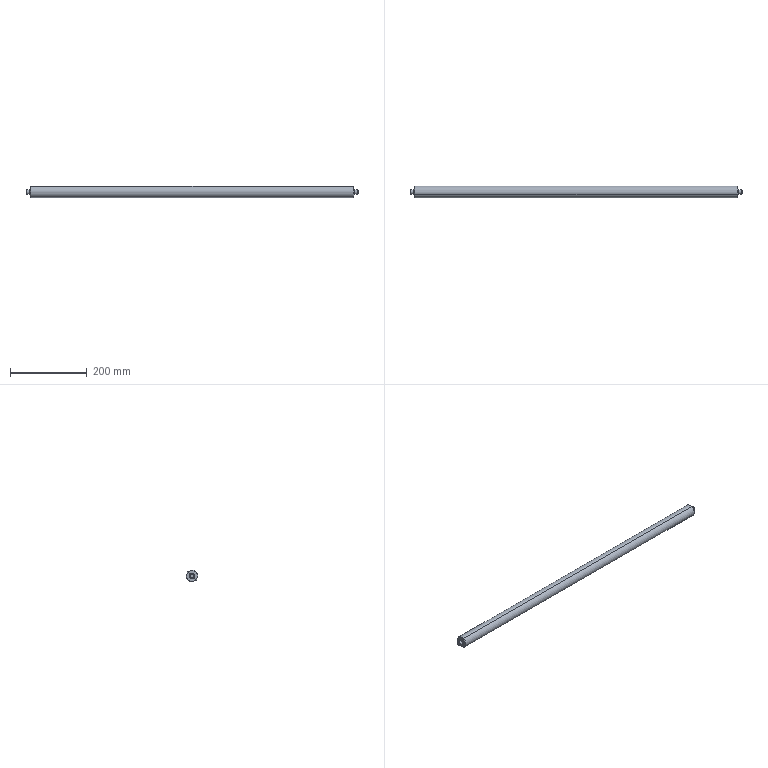Component | SolidWorks | DrivenAxis-1_MainFeedAxis1-1 | 1 solid | 28 faces | box 865 x 30 x 30 mm | volume 598579 mm3 | cone 12 | cylinder 10 | plane 6 | commonest cylinder face diameters 12 x4 15 x4 30 x2
build123d program:
from build123d import *

# Parameters (mm, degrees)
SKETCH1_R           = 15
BOSS_EXTRUDE1_DEPTH = 843
SKETCH3_R           = 7.5
BOSS_EXTRUDE2_DEPTH = 3
BOSS_EXTRUDE3_START = 3
SKETCH4_R           = 7.5
BOSS_EXTRUDE3_DEPTH = 3
SKETCH5_R           = 6
BOSS_EXTRUDE4_DEPTH = 8
BOSS_EXTRUDE5_START = 8
SKETCH6_R           = 6
BOSS_EXTRUDE5_DEPTH = 8
CHAMFER1_SIZE       = 1
CHAMFER2_SIZE       = 1


with BuildPart() as part:
    # Sketch1 → Boss-Extrude1 (new body)
    with BuildSketch(Plane.XY):
        with Locations(Location((0, 0, 0), (0, 0, 180))):
            Circle(SKETCH1_R)
    extrude(amount=BOSS_EXTRUDE1_DEPTH)

    # Sketch3 → Boss-Extrude2 (add)
    with BuildSketch(Plane.XY.offset(843)):
        Circle(SKETCH3_R)
    extrude(amount=BOSS_EXTRUDE2_DEPTH)

    # Sketch4 → Boss-Extrude3 (add)
    with BuildSketch(Plane(origin=(0, 0, 0), x_dir=(-1, 0, 0), z_dir=(0, 0, -1)).offset(BOSS_EXTRUDE3_START)):
        with Locations(Location((0, 0, 0), (0, 0, 180))):
            Circle(SKETCH4_R)
    extrude(amount=-BOSS_EXTRUDE3_DEPTH)

    # Sketch5 → Boss-Extrude4 (add)
    with BuildSketch(Plane(origin=(0, 0, -3), x_dir=(-1, 0, 0), z_dir=(0, 0, -1))):
        Circle(SKETCH5_R)
    extrude(amount=BOSS_EXTRUDE4_DEPTH)

    # Sketch6 → Boss-Extrude5 (add)
    with BuildSketch(Plane.XY.offset(846).offset(BOSS_EXTRUDE5_START)):
        with Locations(Location((0, 0, 0), (0, 0, 180))):
            Circle(SKETCH6_R)
    extrude(amount=-BOSS_EXTRUDE5_DEPTH)

    # Chamfer1
    chamfer1_edges = [part.edges().sort_by_distance(p)[0] for p in [
        (6, 0, 854),
        (15, 0, 843),
        (-7.5, 0, 846),
    ]]
    chamfer(chamfer1_edges, length=CHAMFER1_SIZE)

    # Chamfer2
    chamfer2_edges = [part.edges().sort_by_distance(p)[0] for p in [
        (-7.5, 0, -3),
        (6, 0, -11),
        (15, 0, 0),
    ]]
    chamfer(chamfer2_edges, length=CHAMFER2_SIZE)


solid = part.part

# Placed as in the assembly
solid = solid.moved(Location((13, -30, -174.268), (0, 90, 0)))
STEP:
#1=COLOUR_RGB('',0.7922,0.8196,0.9333);
#2=FILL_AREA_STYLE_COLOUR('',#1);
#3=FILL_AREA_STYLE('',(#2));
#4=SURFACE_STYLE_FILL_AREA(#3);
#5=SURFACE_SIDE_STYLE('',(#4));
#6=SURFACE_STYLE_USAGE(.BOTH.,#5);
#7=PRESENTATION_STYLE_ASSIGNMENT((#6));
#8=CARTESIAN_POINT('',(33.701,-0.9596,-7.366));
#9=VERTEX_POINT('',#8);
#10=CARTESIAN_POINT('',(33.701,-1.403,-6.356));
#11=VERTEX_POINT('',#10);
#12=CARTESIAN_POINT('',(33.701,-1.181,-6.861));
#13=DIRECTION('',(1.,-0.,-0.));
#14=DIRECTION('',(0.,-0.402,0.9157));
#15=AXIS2_PLACEMENT_3D('',#12,#13,#14);
#16=CIRCLE('',#15,0.5512);
#17=EDGE_CURVE('',#9,#11,#16,.T.);
#18=ORIENTED_EDGE('',*,*,#17,.F.);
#19=CARTESIAN_POINT('',(33.661,-0.9437,-7.402));
#20=VERTEX_POINT('',#19);
#21=CARTESIAN_POINT('',(33.661,-0.9437,-7.402));
#22=DIRECTION('',(-0.7071,0.2842,-0.6475));
#23=VECTOR('',#22,39.37);
#24=LINE('',#21,#23);
#25=EDGE_CURVE('',#9,#20,#24,.T.);
#26=ORIENTED_EDGE('',*,*,#25,.T.);
#27=CARTESIAN_POINT('',(33.661,-1.418,-6.32));
#28=VERTEX_POINT('',#27);
#29=CARTESIAN_POINT('',(33.661,-1.181,-6.861));
#30=DIRECTION('',(-1.,0.,0.));
#31=DIRECTION('',(0.,-0.402,0.9157));
#32=AXIS2_PLACEMENT_3D('',#29,#30,#31);
#33=CIRCLE('',#32,0.5906);
#34=EDGE_CURVE('',#28,#20,#33,.T.);
#35=ORIENTED_EDGE('',*,*,#34,.F.);
#36=CARTESIAN_POINT('',(33.661,-1.418,-6.32));
#37=DIRECTION('',(-0.7071,-0.2842,0.6475));
#38=VECTOR('',#37,39.37);
#39=LINE('',#36,#38);
#40=EDGE_CURVE('',#11,#28,#39,.T.);
#41=ORIENTED_EDGE('',*,*,#40,.F.);
#42=EDGE_LOOP('',(#18,#26,#35,#41));
#43=FACE_OUTER_BOUND('',#42,.T.);
#44=CARTESIAN_POINT('',(33.661,-1.181,-6.861));
#45=DIRECTION('',(-1.,0.,0.));
#46=DIRECTION('',(0.,-0.402,0.9157));
#47=AXIS2_PLACEMENT_3D('',#44,#45,#46);
#48=CONICAL_SURFACE('',#47,0.5906,0.7854);
#49=ADVANCED_FACE('',(#43),#48,.T.);
#50=CARTESIAN_POINT('',(33.819,-1.078,-7.095));
#51=VERTEX_POINT('',#50);
#52=CARTESIAN_POINT('',(33.819,-1.284,-6.627));
#53=VERTEX_POINT('',#52);
#54=CARTESIAN_POINT('',(33.819,-1.181,-6.861));
#55=DIRECTION('',(1.,-0.,-0.));
#56=DIRECTION('',(0.,0.402,-0.9157));
#57=AXIS2_PLACEMENT_3D('',#54,#55,#56);
#58=CIRCLE('',#57,0.2559);
#59=EDGE_CURVE('',#51,#53,#58,.T.);
#60=ORIENTED_EDGE('',*,*,#59,.F.);
#61=CARTESIAN_POINT('',(33.78,-1.062,-7.131));
#62=VERTEX_POINT('',#61);
#63=CARTESIAN_POINT('',(33.819,-1.078,-7.095));
#64=DIRECTION('',(-0.7071,0.2842,-0.6475));
#65=VECTOR('',#64,39.37);
#66=LINE('',#63,#65);
#67=EDGE_CURVE('',#51,#62,#66,.T.);
#68=ORIENTED_EDGE('',*,*,#67,.T.);
#69=CARTESIAN_POINT('',(33.78,-1.3,-6.591));
#70=VERTEX_POINT('',#69);
#71=CARTESIAN_POINT('',(33.78,-1.181,-6.861));
#72=DIRECTION('',(-1.,0.,0.));
#73=DIRECTION('',(0.,0.402,-0.9157));
#74=AXIS2_PLACEMENT_3D('',#71,#72,#73);
#75=CIRCLE('',#74,0.2953);
#76=EDGE_CURVE('',#70,#62,#75,.T.);
#77=ORIENTED_EDGE('',*,*,#76,.F.);
#78=CARTESIAN_POINT('',(33.819,-1.284,-6.627));
#79=DIRECTION('',(-0.7071,-0.2842,0.6475));
#80=VECTOR('',#79,39.37);
#81=LINE('',#78,#80);
#82=EDGE_CURVE('',#53,#70,#81,.T.);
#83=ORIENTED_EDGE('',*,*,#82,.F.);
#84=EDGE_LOOP('',(#60,#68,#77,#83));
#85=FACE_OUTER_BOUND('',#84,.T.);
#86=CARTESIAN_POINT('',(33.819,-1.181,-6.861));
#87=DIRECTION('',(-1.,0.,0.));
#88=DIRECTION('',(0.,-0.402,0.9157));
#89=AXIS2_PLACEMENT_3D('',#86,#87,#88);
#90=CONICAL_SURFACE('',#89,0.2559,0.7854);
#91=ADVANCED_FACE('',(#85),#90,.T.);
#92=CARTESIAN_POINT('',(34.134,-1.102,-7.041));
#93=VERTEX_POINT('',#92);
#94=CARTESIAN_POINT('',(34.134,-1.26,-6.681));
#95=VERTEX_POINT('',#94);
#96=CARTESIAN_POINT('',(34.134,-1.181,-6.861));
#97=DIRECTION('',(1.,-0.,-0.));
#98=DIRECTION('',(0.,0.402,-0.9157));
#99=AXIS2_PLACEMENT_3D('',#96,#97,#98);
#100=CIRCLE('',#99,0.1969);
#101=EDGE_CURVE('',#93,#95,#100,.T.);
#102=ORIENTED_EDGE('',*,*,#101,.F.);
#103=CARTESIAN_POINT('',(34.094,-1.086,-7.077));
#104=VERTEX_POINT('',#103);
#105=CARTESIAN_POINT('',(34.134,-1.102,-7.041));
#106=DIRECTION('',(-0.7071,0.2842,-0.6475));
#107=VECTOR('',#106,39.37);
#108=LINE('',#105,#107);
#109=EDGE_CURVE('',#93,#104,#108,.T.);
#110=ORIENTED_EDGE('',*,*,#109,.T.);
#111=CARTESIAN_POINT('',(34.094,-1.276,-6.645));
#112=VERTEX_POINT('',#111);
#113=CARTESIAN_POINT('',(34.094,-1.181,-6.861));
#114=DIRECTION('',(-1.,0.,0.));
#115=DIRECTION('',(0.,0.402,-0.9157));
#116=AXIS2_PLACEMENT_3D('',#113,#114,#115);
#117=CIRCLE('',#116,0.2362);
#118=EDGE_CURVE('',#112,#104,#117,.T.);
#119=ORIENTED_EDGE('',*,*,#118,.F.);
#120=CARTESIAN_POINT('',(34.134,-1.26,-6.681));
#121=DIRECTION('',(-0.7071,-0.2842,0.6475));
#122=VECTOR('',#121,39.37);
#123=LINE('',#120,#122);
#124=EDGE_CURVE('',#95,#112,#123,.T.);
#125=ORIENTED_EDGE('',*,*,#124,.F.);
#126=EDGE_LOOP('',(#102,#110,#119,#125));
#127=FACE_OUTER_BOUND('',#126,.T.);
#128=CARTESIAN_POINT('',(34.134,-1.181,-6.861));
#129=DIRECTION('',(-1.,0.,0.));
#130=DIRECTION('',(0.,-0.402,0.9157));
#131=AXIS2_PLACEMENT_3D('',#128,#129,#130);
#132=CONICAL_SURFACE('',#131,0.1969,0.7854);
#133=ADVANCED_FACE('',(#127),#132,.T.);
#134=CARTESIAN_POINT('',(0.5118,-1.403,-6.356));
#135=VERTEX_POINT('',#134);
#136=CARTESIAN_POINT('',(0.5118,-0.9596,-7.366));
#137=VERTEX_POINT('',#136);
#138=CARTESIAN_POINT('',(0.5118,-1.181,-6.861));
#139=DIRECTION('',(-1.,0.,0.));
#140=DIRECTION('',(0.,-0.402,0.9157));
#141=AXIS2_PLACEMENT_3D('',#138,#139,#140);
#142=CIRCLE('',#141,0.5512);
#143=EDGE_CURVE('',#135,#137,#142,.T.);
#144=ORIENTED_EDGE('',*,*,#143,.F.);
#145=CARTESIAN_POINT('',(0.5512,-1.418,-6.32));
#146=VERTEX_POINT('',#145);
#147=CARTESIAN_POINT('',(0.5118,-1.403,-6.356));
#148=DIRECTION('',(0.7071,-0.2842,0.6475));
#149=VECTOR('',#148,39.37);
#150=LINE('',#147,#149);
#151=EDGE_CURVE('',#135,#146,#150,.T.);
#152=ORIENTED_EDGE('',*,*,#151,.T.);
#153=CARTESIAN_POINT('',(0.5512,-0.9437,-7.402));
#154=VERTEX_POINT('',#153);
#155=CARTESIAN_POINT('',(0.5512,-1.181,-6.861));
#156=DIRECTION('',(1.,-0.,-0.));
#157=DIRECTION('',(0.,-0.402,0.9157));
#158=AXIS2_PLACEMENT_3D('',#155,#156,#157);
#159=CIRCLE('',#158,0.5906);
#160=EDGE_CURVE('',#154,#146,#159,.T.);
#161=ORIENTED_EDGE('',*,*,#160,.F.);
#162=CARTESIAN_POINT('',(0.5118,-0.9596,-7.366));
#163=DIRECTION('',(0.7071,0.2842,-0.6475));
#164=VECTOR('',#163,39.37);
#165=LINE('',#162,#164);
#166=EDGE_CURVE('',#137,#154,#165,.T.);
#167=ORIENTED_EDGE('',*,*,#166,.F.);
#168=EDGE_LOOP('',(#144,#152,#161,#167));
#169=FACE_OUTER_BOUND('',#168,.T.);
#170=CARTESIAN_POINT('',(0.5118,-1.181,-6.861));
#171=DIRECTION('',(1.,-0.,-0.));
#172=DIRECTION('',(-0.,0.402,-0.9157));
#173=AXIS2_PLACEMENT_3D('',#170,#171,#172);
#174=CONICAL_SURFACE('',#173,0.5512,0.7854);
#175=ADVANCED_FACE('',(#169),#174,.T.);
#176=CARTESIAN_POINT('',(0.3937,-1.284,-6.627));
#177=VERTEX_POINT('',#176);
#178=CARTESIAN_POINT('',(0.3937,-1.078,-7.095));
#179=VERTEX_POINT('',#178);
#180=CARTESIAN_POINT('',(0.3937,-1.181,-6.861));
#181=DIRECTION('',(-1.,0.,0.));
#182=DIRECTION('',(0.,-0.402,0.9157));
#183=AXIS2_PLACEMENT_3D('',#180,#181,#182);
#184=CIRCLE('',#183,0.2559);
#185=EDGE_CURVE('',#177,#179,#184,.T.);
#186=ORIENTED_EDGE('',*,*,#185,.F.);
#187=CARTESIAN_POINT('',(0.4331,-1.3,-6.591));
#188=VERTEX_POINT('',#187);
#189=CARTESIAN_POINT('',(0.3937,-1.284,-6.627));
#190=DIRECTION('',(0.7071,-0.2842,0.6475));
#191=VECTOR('',#190,39.37);
#192=LINE('',#189,#191);
#193=EDGE_CURVE('',#177,#188,#192,.T.);
#194=ORIENTED_EDGE('',*,*,#193,.T.);
#195=CARTESIAN_POINT('',(0.4331,-1.062,-7.131));
#196=VERTEX_POINT('',#195);
#197=CARTESIAN_POINT('',(0.4331,-1.181,-6.861));
#198=DIRECTION('',(1.,-0.,-0.));
#199=DIRECTION('',(0.,-0.402,0.9157));
#200=AXIS2_PLACEMENT_3D('',#197,#198,#199);
#201=CIRCLE('',#200,0.2953);
#202=EDGE_CURVE('',#196,#188,#201,.T.);
#203=ORIENTED_EDGE('',*,*,#202,.F.);
#204=CARTESIAN_POINT('',(0.3937,-1.078,-7.095));
#205=DIRECTION('',(0.7071,0.2842,-0.6475));
#206=VECTOR('',#205,39.37);
#207=LINE('',#204,#206);
#208=EDGE_CURVE('',#179,#196,#207,.T.);
#209=ORIENTED_EDGE('',*,*,#208,.F.);
#210=EDGE_LOOP('',(#186,#194,#203,#209));
#211=FACE_OUTER_BOUND('',#210,.T.);
#212=CARTESIAN_POINT('',(0.3937,-1.181,-6.861));
#213=DIRECTION('',(1.,-0.,-0.));
#214=DIRECTION('',(-0.,0.402,-0.9157));
#215=AXIS2_PLACEMENT_3D('',#212,#213,#214);
#216=CONICAL_SURFACE('',#215,0.2559,0.7854);
#217=ADVANCED_FACE('',(#211),#216,.T.);
#218=CARTESIAN_POINT('',(0.07874,-1.26,-6.681));
#219=VERTEX_POINT('',#218);
#220=CARTESIAN_POINT('',(0.07874,-1.102,-7.041));
#221=VERTEX_POINT('',#220);
#222=CARTESIAN_POINT('',(0.07874,-1.181,-6.861));
#223=DIRECTION('',(-1.,0.,0.));
#224=DIRECTION('',(0.,-0.402,0.9157));
#225=AXIS2_PLACEMENT_3D('',#222,#223,#224);
#226=CIRCLE('',#225,0.1969);
#227=EDGE_CURVE('',#219,#221,#226,.T.);
#228=ORIENTED_EDGE('',*,*,#227,.F.);
#229=CARTESIAN_POINT('',(0.1181,-1.276,-6.645));
#230=VERTEX_POINT('',#229);
#231=CARTESIAN_POINT('',(0.07874,-1.26,-6.681));
#232=DIRECTION('',(0.7071,-0.2842,0.6475));
#233=VECTOR('',#232,39.37);
#234=LINE('',#231,#233);
#235=EDGE_CURVE('',#219,#230,#234,.T.);
#236=ORIENTED_EDGE('',*,*,#235,.T.);
#237=CARTESIAN_POINT('',(0.1181,-1.086,-7.077));
#238=VERTEX_POINT('',#237);
#239=CARTESIAN_POINT('',(0.1181,-1.181,-6.861));
#240=DIRECTION('',(1.,-0.,-0.));
#241=DIRECTION('',(0.,-0.402,0.9157));
#242=AXIS2_PLACEMENT_3D('',#239,#240,#241);
#243=CIRCLE('',#242,0.2362);
#244=EDGE_CURVE('',#238,#230,#243,.T.);
#245=ORIENTED_EDGE('',*,*,#244,.F.);
#246=CARTESIAN_POINT('',(0.07874,-1.102,-7.041));
#247=DIRECTION('',(0.7071,0.2842,-0.6475));
#248=VECTOR('',#247,39.37);
#249=LINE('',#246,#248);
#250=EDGE_CURVE('',#221,#238,#249,.T.);
#251=ORIENTED_EDGE('',*,*,#250,.F.);
#252=EDGE_LOOP('',(#228,#236,#245,#251));
#253=FACE_OUTER_BOUND('',#252,.T.);
#254=CARTESIAN_POINT('',(0.07874,-1.181,-6.861));
#255=DIRECTION('',(1.,-0.,-0.));
#256=DIRECTION('',(-0.,0.402,-0.9157));
#257=AXIS2_PLACEMENT_3D('',#254,#255,#256);
#258=CONICAL_SURFACE('',#257,0.1969,0.7854);
#259=ADVANCED_FACE('',(#253),#258,.T.);
#260=ORIENTED_EDGE('',*,*,#244,.T.);
#261=CARTESIAN_POINT('',(0.3937,-1.276,-6.645));
#262=VERTEX_POINT('',#261);
#263=CARTESIAN_POINT('',(0.07874,-1.276,-6.645));
#264=DIRECTION('',(1.,-0.,-0.));
#265=VECTOR('',#264,39.37);
#266=LINE('',#263,#265);
#267=EDGE_CURVE('',#230,#262,#266,.T.);
#268=ORIENTED_EDGE('',*,*,#267,.T.);
#269=CARTESIAN_POINT('',(0.3937,-1.086,-7.077));
#270=VERTEX_POINT('',#269);
#271=CARTESIAN_POINT('',(0.3937,-1.181,-6.861));
#272=DIRECTION('',(-1.,0.,0.));
#273=DIRECTION('',(0.,-0.402,0.9157));
#274=AXIS2_PLACEMENT_3D('',#271,#272,#273);
#275=CIRCLE('',#274,0.2362);
#276=EDGE_CURVE('',#262,#270,#275,.T.);
#277=ORIENTED_EDGE('',*,*,#276,.T.);
#278=CARTESIAN_POINT('',(0.07874,-1.086,-7.077));
#279=DIRECTION('',(1.,-0.,-0.));
#280=VECTOR('',#279,39.37);
#281=LINE('',#278,#280);
#282=EDGE_CURVE('',#238,#270,#281,.T.);
#283=ORIENTED_EDGE('',*,*,#282,.F.);
#284=EDGE_LOOP('',(#260,#268,#277,#283));
#285=FACE_OUTER_BOUND('',#284,.T.);
#286=CARTESIAN_POINT('',(0.07874,-1.181,-6.861));
#287=DIRECTION('',(1.,-0.,-0.));
#288=DIRECTION('',(-0.,0.402,-0.9157));
#289=AXIS2_PLACEMENT_3D('',#286,#287,#288);
#290=CYLINDRICAL_SURFACE('',#289,0.2362);
#291=ADVANCED_FACE('',(#285),#290,.T.);
#292=ORIENTED_EDGE('',*,*,#118,.T.);
#293=CARTESIAN_POINT('',(33.819,-1.086,-7.077));
#294=VERTEX_POINT('',#293);
#295=CARTESIAN_POINT('',(34.134,-1.086,-7.077));
#296=DIRECTION('',(-1.,0.,0.));
#297=VECTOR('',#296,39.37);
#298=LINE('',#295,#297);
#299=EDGE_CURVE('',#104,#294,#298,.T.);
#300=ORIENTED_EDGE('',*,*,#299,.T.);
#301=CARTESIAN_POINT('',(33.819,-1.276,-6.645));
#302=VERTEX_POINT('',#301);
#303=CARTESIAN_POINT('',(33.819,-1.181,-6.861));
#304=DIRECTION('',(1.,-0.,-0.));
#305=DIRECTION('',(0.,0.402,-0.9157));
#306=AXIS2_PLACEMENT_3D('',#303,#304,#305);
#307=CIRCLE('',#306,0.2362);
#308=EDGE_CURVE('',#294,#302,#307,.T.);
#309=ORIENTED_EDGE('',*,*,#308,.T.);
#310=CARTESIAN_POINT('',(34.134,-1.276,-6.645));
#311=DIRECTION('',(-1.,0.,0.));
#312=VECTOR('',#311,39.37);
#313=LINE('',#310,#312);
#314=EDGE_CURVE('',#112,#302,#313,.T.);
#315=ORIENTED_EDGE('',*,*,#314,.F.);
#316=EDGE_LOOP('',(#292,#300,#309,#315));
#317=FACE_OUTER_BOUND('',#316,.T.);
#318=CARTESIAN_POINT('',(34.134,-1.181,-6.861));
#319=DIRECTION('',(-1.,0.,0.));
#320=DIRECTION('',(0.,-0.402,0.9157));
#321=AXIS2_PLACEMENT_3D('',#318,#319,#320);
#322=CYLINDRICAL_SURFACE('',#321,0.2362);
#323=ADVANCED_FACE('',(#317),#322,.T.);
#324=ORIENTED_EDGE('',*,*,#76,.T.);
#325=CARTESIAN_POINT('',(33.701,-1.062,-7.131));
#326=VERTEX_POINT('',#325);
#327=CARTESIAN_POINT('',(33.819,-1.062,-7.131));
#328=DIRECTION('',(-1.,0.,0.));
#329=VECTOR('',#328,39.37);
#330=LINE('',#327,#329);
#331=EDGE_CURVE('',#62,#326,#330,.T.);
#332=ORIENTED_EDGE('',*,*,#331,.T.);
#333=CARTESIAN_POINT('',(33.701,-1.3,-6.591));
#334=VERTEX_POINT('',#333);
#335=CARTESIAN_POINT('',(33.701,-1.181,-6.861));
#336=DIRECTION('',(1.,-0.,-0.));
#337=DIRECTION('',(0.,-0.402,0.9157));
#338=AXIS2_PLACEMENT_3D('',#335,#336,#337);
#339=CIRCLE('',#338,0.2953);
#340=EDGE_CURVE('',#326,#334,#339,.T.);
#341=ORIENTED_EDGE('',*,*,#340,.T.);
#342=CARTESIAN_POINT('',(33.819,-1.3,-6.591));
#343=DIRECTION('',(-1.,0.,0.));
#344=VECTOR('',#343,39.37);
#345=LINE('',#342,#344);
#346=EDGE_CURVE('',#70,#334,#345,.T.);
#347=ORIENTED_EDGE('',*,*,#346,.F.);
#348=EDGE_LOOP('',(#324,#332,#341,#347));
#349=FACE_OUTER_BOUND('',#348,.T.);
#350=CARTESIAN_POINT('',(33.819,-1.181,-6.861));
#351=DIRECTION('',(-1.,0.,0.));
#352=DIRECTION('',(0.,-0.402,0.9157));
#353=AXIS2_PLACEMENT_3D('',#350,#351,#352);
#354=CYLINDRICAL_SURFACE('',#353,0.2953);
#355=ADVANCED_FACE('',(#349),#354,.T.);
#356=ORIENTED_EDGE('',*,*,#202,.T.);
#357=CARTESIAN_POINT('',(0.5118,-1.3,-6.591));
#358=VERTEX_POINT('',#357);
#359=CARTESIAN_POINT('',(0.3937,-1.3,-6.591));
#360=DIRECTION('',(1.,-0.,-0.));
#361=VECTOR('',#360,39.37);
#362=LINE('',#359,#361);
#363=EDGE_CURVE('',#188,#358,#362,.T.);
#364=ORIENTED_EDGE('',*,*,#363,.T.);
#365=CARTESIAN_POINT('',(0.5118,-1.062,-7.131));
#366=VERTEX_POINT('',#365);
#367=CARTESIAN_POINT('',(0.5118,-1.181,-6.861));
#368=DIRECTION('',(-1.,0.,0.));
#369=DIRECTION('',(0.,-0.402,0.9157));
#370=AXIS2_PLACEMENT_3D('',#367,#368,#369);
#371=CIRCLE('',#370,0.2953);
#372=EDGE_CURVE('',#358,#366,#371,.T.);
#373=ORIENTED_EDGE('',*,*,#372,.T.);
#374=CARTESIAN_POINT('',(0.3937,-1.062,-7.131));
#375=DIRECTION('',(1.,-0.,-0.));
#376=VECTOR('',#375,39.37);
#377=LINE('',#374,#376);
#378=EDGE_CURVE('',#196,#366,#377,.T.);
#379=ORIENTED_EDGE('',*,*,#378,.F.);
#380=EDGE_LOOP('',(#356,#364,#373,#379));
#381=FACE_OUTER_BOUND('',#380,.T.);
#382=CARTESIAN_POINT('',(0.3937,-1.181,-6.861));
#383=DIRECTION('',(1.,-0.,-0.));
#384=DIRECTION('',(-0.,0.402,-0.9157));
#385=AXIS2_PLACEMENT_3D('',#382,#383,#384);
#386=CYLINDRICAL_SURFACE('',#385,0.2953);
#387=ADVANCED_FACE('',(#381),#386,.T.);
#388=ORIENTED_EDGE('',*,*,#160,.T.);
#389=CARTESIAN_POINT('',(0.5118,-1.418,-6.32));
#390=DIRECTION('',(1.,-0.,-0.));
#391=VECTOR('',#390,39.37);
#392=LINE('',#389,#391);
#393=EDGE_CURVE('',#146,#28,#392,.T.);
#394=ORIENTED_EDGE('',*,*,#393,.T.);
#395=ORIENTED_EDGE('',*,*,#34,.T.);
#396=CARTESIAN_POINT('',(0.5118,-0.9437,-7.402));
#397=DIRECTION('',(1.,-0.,-0.));
#398=VECTOR('',#397,39.37);
#399=LINE('',#396,#398);
#400=EDGE_CURVE('',#154,#20,#399,.T.);
#401=ORIENTED_EDGE('',*,*,#400,.F.);
#402=EDGE_LOOP('',(#388,#394,#395,#401));
#403=FACE_OUTER_BOUND('',#402,.T.);
#404=CARTESIAN_POINT('',(0.5118,-1.181,-6.861));
#405=DIRECTION('',(1.,-0.,-0.));
#406=DIRECTION('',(-0.,0.402,-0.9157));
#407=AXIS2_PLACEMENT_3D('',#404,#405,#406);
#408=CYLINDRICAL_SURFACE('',#407,0.5906);
#409=ADVANCED_FACE('',(#403),#408,.T.);
#410=ORIENTED_EDGE('',*,*,#393,.F.);
#411=CARTESIAN_POINT('',(0.5512,-1.181,-6.861));
#412=DIRECTION('',(1.,-0.,-0.));
#413=DIRECTION('',(0.,-0.402,0.9157));
#414=AXIS2_PLACEMENT_3D('',#411,#412,#413);
#415=CIRCLE('',#414,0.5906);
#416=EDGE_CURVE('',#146,#154,#415,.T.);
#417=ORIENTED_EDGE('',*,*,#416,.T.);
#418=ORIENTED_EDGE('',*,*,#400,.T.);
#419=CARTESIAN_POINT('',(33.661,-1.181,-6.861));
#420=DIRECTION('',(-1.,0.,0.));
#421=DIRECTION('',(0.,-0.402,0.9157));
#422=AXIS2_PLACEMENT_3D('',#419,#420,#421);
#423=CIRCLE('',#422,0.5906);
#424=EDGE_CURVE('',#20,#28,#423,.T.);
#425=ORIENTED_EDGE('',*,*,#424,.T.);
#426=EDGE_LOOP('',(#410,#417,#418,#425));
#427=FACE_OUTER_BOUND('',#426,.T.);
#428=CARTESIAN_POINT('',(0.5118,-1.181,-6.861));
#429=DIRECTION('',(1.,-0.,-0.));
#430=DIRECTION('',(-0.,0.402,-0.9157));
#431=AXIS2_PLACEMENT_3D('',#428,#429,#430);
#432=CYLINDRICAL_SURFACE('',#431,0.5906);
#433=ADVANCED_FACE('',(#427),#432,.T.);
#434=CARTESIAN_POINT('',(0.5118,-1.181,-6.861));
#435=DIRECTION('',(-1.,0.,0.));
#436=DIRECTION('',(0.,-0.402,0.9157));
#437=AXIS2_PLACEMENT_3D('',#434,#435,#436);
#438=CIRCLE('',#437,0.5512);
#439=EDGE_CURVE('',#137,#135,#438,.T.);
#440=ORIENTED_EDGE('',*,*,#439,.T.);
#441=ORIENTED_EDGE('',*,*,#143,.T.);
#442=EDGE_LOOP('',(#440,#441));
#443=FACE_OUTER_BOUND('',#442,.T.);
#444=CARTESIAN_POINT('',(0.5118,-1.181,-6.861));
#445=DIRECTION('',(-1.,0.,0.));
#446=DIRECTION('',(0.,-0.402,0.9157));
#447=AXIS2_PLACEMENT_3D('',#444,#445,#446);
#448=CIRCLE('',#447,0.2953);
#449=EDGE_CURVE('',#366,#358,#448,.T.);
#450=ORIENTED_EDGE('',*,*,#449,.F.);
#451=ORIENTED_EDGE('',*,*,#372,.F.);
#452=EDGE_LOOP('',(#450,#451));
#453=FACE_BOUND('',#452,.T.);
#454=CARTESIAN_POINT('',(0.5118,-1.181,-6.861));
#455=DIRECTION('',(-1.,0.,0.));
#456=DIRECTION('',(0.,-0.402,0.9157));
#457=AXIS2_PLACEMENT_3D('',#454,#455,#456);
#458=PLANE('',#457);
#459=ADVANCED_FACE('',(#443,#453),#458,.T.);
#460=CARTESIAN_POINT('',(33.701,-1.181,-6.861));
#461=DIRECTION('',(1.,-0.,-0.));
#462=DIRECTION('',(0.,-0.402,0.9157));
#463=AXIS2_PLACEMENT_3D('',#460,#461,#462);
#464=CIRCLE('',#463,0.5512);
#465=EDGE_CURVE('',#11,#9,#464,.T.);
#466=ORIENTED_EDGE('',*,*,#465,.T.);
#467=ORIENTED_EDGE('',*,*,#17,.T.);
#468=EDGE_LOOP('',(#466,#467));
#469=FACE_OUTER_BOUND('',#468,.T.);
#470=CARTESIAN_POINT('',(33.701,-1.181,-6.861));
#471=DIRECTION('',(1.,-0.,-0.));
#472=DIRECTION('',(0.,-0.402,0.9157));
#473=AXIS2_PLACEMENT_3D('',#470,#471,#472);
#474=CIRCLE('',#473,0.2953);
#475=EDGE_CURVE('',#334,#326,#474,.T.);
#476=ORIENTED_EDGE('',*,*,#475,.F.);
#477=ORIENTED_EDGE('',*,*,#340,.F.);
#478=EDGE_LOOP('',(#476,#477));
#479=FACE_BOUND('',#478,.T.);
#480=CARTESIAN_POINT('',(33.701,-1.181,-6.861));
#481=DIRECTION('',(-1.,0.,0.));
#482=DIRECTION('',(0.,-0.402,0.9157));
#483=AXIS2_PLACEMENT_3D('',#480,#481,#482);
#484=PLANE('',#483);
#485=ADVANCED_FACE('',(#469,#479),#484,.F.);
#486=ORIENTED_EDGE('',*,*,#363,.F.);
#487=CARTESIAN_POINT('',(0.4331,-1.181,-6.861));
#488=DIRECTION('',(1.,-0.,-0.));
#489=DIRECTION('',(0.,-0.402,0.9157));
#490=AXIS2_PLACEMENT_3D('',#487,#488,#489);
#491=CIRCLE('',#490,0.2953);
#492=EDGE_CURVE('',#188,#196,#491,.T.);
#493=ORIENTED_EDGE('',*,*,#492,.T.);
#494=ORIENTED_EDGE('',*,*,#378,.T.);
#495=ORIENTED_EDGE('',*,*,#449,.T.);
#496=EDGE_LOOP('',(#486,#493,#494,#495));
#497=FACE_OUTER_BOUND('',#496,.T.);
#498=CARTESIAN_POINT('',(0.3937,-1.181,-6.861));
#499=DIRECTION('',(1.,-0.,-0.));
#500=DIRECTION('',(-0.,0.402,-0.9157));
#501=AXIS2_PLACEMENT_3D('',#498,#499,#500);
#502=CYLINDRICAL_SURFACE('',#501,0.2953);
#503=ADVANCED_FACE('',(#497),#502,.T.);
#504=CARTESIAN_POINT('',(0.3937,-1.181,-6.861));
#505=DIRECTION('',(-1.,0.,0.));
#506=DIRECTION('',(0.,-0.402,0.9157));
#507=AXIS2_PLACEMENT_3D('',#504,#505,#506);
#508=CIRCLE('',#507,0.2559);
#509=EDGE_CURVE('',#179,#177,#508,.T.);
#510=ORIENTED_EDGE('',*,*,#509,.T.);
#511=ORIENTED_EDGE('',*,*,#185,.T.);
#512=EDGE_LOOP('',(#510,#511));
#513=FACE_OUTER_BOUND('',#512,.T.);
#514=CARTESIAN_POINT('',(0.3937,-1.181,-6.861));
#515=DIRECTION('',(-1.,0.,0.));
#516=DIRECTION('',(0.,-0.402,0.9157));
#517=AXIS2_PLACEMENT_3D('',#514,#515,#516);
#518=CIRCLE('',#517,0.2362);
#519=EDGE_CURVE('',#270,#262,#518,.T.);
#520=ORIENTED_EDGE('',*,*,#519,.F.);
#521=ORIENTED_EDGE('',*,*,#276,.F.);
#522=EDGE_LOOP('',(#520,#521));
#523=FACE_BOUND('',#522,.T.);
#524=CARTESIAN_POINT('',(0.3937,-1.181,-6.861));
#525=DIRECTION('',(-1.,0.,0.));
#526=DIRECTION('',(0.,-0.402,0.9157));
#527=AXIS2_PLACEMENT_3D('',#524,#525,#526);
#528=PLANE('',#527);
#529=ADVANCED_FACE('',(#513,#523),#528,.T.);
#530=ORIENTED_EDGE('',*,*,#331,.F.);
#531=CARTESIAN_POINT('',(33.78,-1.181,-6.861));
#532=DIRECTION('',(-1.,0.,0.));
#533=DIRECTION('',(0.,0.402,-0.9157));
#534=AXIS2_PLACEMENT_3D('',#531,#532,#533);
#535=CIRCLE('',#534,0.2953);
#536=EDGE_CURVE('',#62,#70,#535,.T.);
#537=ORIENTED_EDGE('',*,*,#536,.T.);
#538=ORIENTED_EDGE('',*,*,#346,.T.);
#539=ORIENTED_EDGE('',*,*,#475,.T.);
#540=EDGE_LOOP('',(#530,#537,#538,#539));
#541=FACE_OUTER_BOUND('',#540,.T.);
#542=CARTESIAN_POINT('',(33.819,-1.181,-6.861));
#543=DIRECTION('',(-1.,0.,0.));
#544=DIRECTION('',(0.,-0.402,0.9157));
#545=AXIS2_PLACEMENT_3D('',#542,#543,#544);
#546=CYLINDRICAL_SURFACE('',#545,0.2953);
#547=ADVANCED_FACE('',(#541),#546,.T.);
#548=CARTESIAN_POINT('',(33.819,-1.181,-6.861));
#549=DIRECTION('',(1.,-0.,-0.));
#550=DIRECTION('',(0.,0.402,-0.9157));
#551=AXIS2_PLACEMENT_3D('',#548,#549,#550);
#552=CIRCLE('',#551,0.2559);
#553=EDGE_CURVE('',#53,#51,#552,.T.);
#554=ORIENTED_EDGE('',*,*,#553,.T.);
#555=ORIENTED_EDGE('',*,*,#59,.T.);
#556=EDGE_LOOP('',(#554,#555));
#557=FACE_OUTER_BOUND('',#556,.T.);
#558=CARTESIAN_POINT('',(33.819,-1.181,-6.861));
#559=DIRECTION('',(1.,-0.,-0.));
#560=DIRECTION('',(0.,0.402,-0.9157));
#561=AXIS2_PLACEMENT_3D('',#558,#559,#560);
#562=CIRCLE('',#561,0.2362);
#563=EDGE_CURVE('',#302,#294,#562,.T.);
#564=ORIENTED_EDGE('',*,*,#563,.F.);
#565=ORIENTED_EDGE('',*,*,#308,.F.);
#566=EDGE_LOOP('',(#564,#565));
#567=FACE_BOUND('',#566,.T.);
#568=CARTESIAN_POINT('',(33.819,-1.181,-6.861));
#569=DIRECTION('',(1.,-0.,-0.));
#570=DIRECTION('',(-0.,0.402,-0.9157));
#571=AXIS2_PLACEMENT_3D('',#568,#569,#570);
#572=PLANE('',#571);
#573=ADVANCED_FACE('',(#557,#567),#572,.T.);
#574=ORIENTED_EDGE('',*,*,#299,.F.);
#575=CARTESIAN_POINT('',(34.094,-1.181,-6.861));
#576=DIRECTION('',(-1.,0.,0.));
#577=DIRECTION('',(0.,0.402,-0.9157));
#578=AXIS2_PLACEMENT_3D('',#575,#576,#577);
#579=CIRCLE('',#578,0.2362);
#580=EDGE_CURVE('',#104,#112,#579,.T.);
#581=ORIENTED_EDGE('',*,*,#580,.T.);
#582=ORIENTED_EDGE('',*,*,#314,.T.);
#583=ORIENTED_EDGE('',*,*,#563,.T.);
#584=EDGE_LOOP('',(#574,#581,#582,#583));
#585=FACE_OUTER_BOUND('',#584,.T.);
#586=CARTESIAN_POINT('',(34.134,-1.181,-6.861));
#587=DIRECTION('',(-1.,0.,0.));
#588=DIRECTION('',(0.,-0.402,0.9157));
#589=AXIS2_PLACEMENT_3D('',#586,#587,#588);
#590=CYLINDRICAL_SURFACE('',#589,0.2362);
#591=ADVANCED_FACE('',(#585),#590,.T.);
#592=CARTESIAN_POINT('',(34.134,-1.181,-6.861));
#593=DIRECTION('',(1.,-0.,-0.));
#594=DIRECTION('',(0.,0.402,-0.9157));
#595=AXIS2_PLACEMENT_3D('',#592,#593,#594);
#596=CIRCLE('',#595,0.1969);
#597=EDGE_CURVE('',#95,#93,#596,.T.);
#598=ORIENTED_EDGE('',*,*,#597,.T.);
#599=ORIENTED_EDGE('',*,*,#101,.T.);
#600=EDGE_LOOP('',(#598,#599));
#601=FACE_OUTER_BOUND('',#600,.T.);
#602=CARTESIAN_POINT('',(34.134,-1.181,-6.861));
#603=DIRECTION('',(1.,-0.,-0.));
#604=DIRECTION('',(-0.,0.402,-0.9157));
#605=AXIS2_PLACEMENT_3D('',#602,#603,#604);
#606=PLANE('',#605);
#607=ADVANCED_FACE('',(#601),#606,.T.);
#608=ORIENTED_EDGE('',*,*,#267,.F.);
#609=CARTESIAN_POINT('',(0.1181,-1.181,-6.861));
#610=DIRECTION('',(1.,-0.,-0.));
#611=DIRECTION('',(0.,-0.402,0.9157));
#612=AXIS2_PLACEMENT_3D('',#609,#610,#611);
#613=CIRCLE('',#612,0.2362);
#614=EDGE_CURVE('',#230,#238,#613,.T.);
#615=ORIENTED_EDGE('',*,*,#614,.T.);
#616=ORIENTED_EDGE('',*,*,#282,.T.);
#617=ORIENTED_EDGE('',*,*,#519,.T.);
#618=EDGE_LOOP('',(#608,#615,#616,#617));
#619=FACE_OUTER_BOUND('',#618,.T.);
#620=CARTESIAN_POINT('',(0.07874,-1.181,-6.861));
#621=DIRECTION('',(1.,-0.,-0.));
#622=DIRECTION('',(-0.,0.402,-0.9157));
#623=AXIS2_PLACEMENT_3D('',#620,#621,#622);
#624=CYLINDRICAL_SURFACE('',#623,0.2362);
#625=ADVANCED_FACE('',(#619),#624,.T.);
#626=CARTESIAN_POINT('',(0.07874,-1.181,-6.861));
#627=DIRECTION('',(-1.,0.,0.));
#628=DIRECTION('',(0.,-0.402,0.9157));
#629=AXIS2_PLACEMENT_3D('',#626,#627,#628);
#630=CIRCLE('',#629,0.1969);
#631=EDGE_CURVE('',#221,#219,#630,.T.);
#632=ORIENTED_EDGE('',*,*,#631,.T.);
#633=ORIENTED_EDGE('',*,*,#227,.T.);
#634=EDGE_LOOP('',(#632,#633));
#635=FACE_OUTER_BOUND('',#634,.T.);
#636=CARTESIAN_POINT('',(0.07874,-1.181,-6.861));
#637=DIRECTION('',(-1.,0.,0.));
#638=DIRECTION('',(0.,-0.402,0.9157));
#639=AXIS2_PLACEMENT_3D('',#636,#637,#638);
#640=PLANE('',#639);
#641=ADVANCED_FACE('',(#635),#640,.T.);
#642=ORIENTED_EDGE('',*,*,#235,.F.);
#643=ORIENTED_EDGE('',*,*,#631,.F.);
#644=ORIENTED_EDGE('',*,*,#250,.T.);
#645=ORIENTED_EDGE('',*,*,#614,.F.);
#646=EDGE_LOOP('',(#642,#643,#644,#645));
#647=FACE_OUTER_BOUND('',#646,.T.);
#648=CARTESIAN_POINT('',(0.07874,-1.181,-6.861));
#649=DIRECTION('',(1.,-0.,-0.));
#650=DIRECTION('',(-0.,0.402,-0.9157));
#651=AXIS2_PLACEMENT_3D('',#648,#649,#650);
#652=CONICAL_SURFACE('',#651,0.1969,0.7854);
#653=ADVANCED_FACE('',(#647),#652,.T.);
#654=ORIENTED_EDGE('',*,*,#193,.F.);
#655=ORIENTED_EDGE('',*,*,#509,.F.);
#656=ORIENTED_EDGE('',*,*,#208,.T.);
#657=ORIENTED_EDGE('',*,*,#492,.F.);
#658=EDGE_LOOP('',(#654,#655,#656,#657));
#659=FACE_OUTER_BOUND('',#658,.T.);
#660=CARTESIAN_POINT('',(0.3937,-1.181,-6.861));
#661=DIRECTION('',(1.,-0.,-0.));
#662=DIRECTION('',(-0.,0.402,-0.9157));
#663=AXIS2_PLACEMENT_3D('',#660,#661,#662);
#664=CONICAL_SURFACE('',#663,0.2559,0.7854);
#665=ADVANCED_FACE('',(#659),#664,.T.);
#666=ORIENTED_EDGE('',*,*,#151,.F.);
#667=ORIENTED_EDGE('',*,*,#439,.F.);
#668=ORIENTED_EDGE('',*,*,#166,.T.);
#669=ORIENTED_EDGE('',*,*,#416,.F.);
#670=EDGE_LOOP('',(#666,#667,#668,#669));
#671=FACE_OUTER_BOUND('',#670,.T.);
#672=CARTESIAN_POINT('',(0.5118,-1.181,-6.861));
#673=DIRECTION('',(1.,-0.,-0.));
#674=DIRECTION('',(-0.,0.402,-0.9157));
#675=AXIS2_PLACEMENT_3D('',#672,#673,#674);
#676=CONICAL_SURFACE('',#675,0.5512,0.7854);
#677=ADVANCED_FACE('',(#671),#676,.T.);
#678=ORIENTED_EDGE('',*,*,#109,.F.);
#679=ORIENTED_EDGE('',*,*,#597,.F.);
#680=ORIENTED_EDGE('',*,*,#124,.T.);
#681=ORIENTED_EDGE('',*,*,#580,.F.);
#682=EDGE_LOOP('',(#678,#679,#680,#681));
#683=FACE_OUTER_BOUND('',#682,.T.);
#684=CARTESIAN_POINT('',(34.134,-1.181,-6.861));
#685=DIRECTION('',(-1.,0.,0.));
#686=DIRECTION('',(0.,-0.402,0.9157));
#687=AXIS2_PLACEMENT_3D('',#684,#685,#686);
#688=CONICAL_SURFACE('',#687,0.1969,0.7854);
#689=ADVANCED_FACE('',(#683),#688,.T.);
#690=ORIENTED_EDGE('',*,*,#67,.F.);
#691=ORIENTED_EDGE('',*,*,#553,.F.);
#692=ORIENTED_EDGE('',*,*,#82,.T.);
#693=ORIENTED_EDGE('',*,*,#536,.F.);
#694=EDGE_LOOP('',(#690,#691,#692,#693));
#695=FACE_OUTER_BOUND('',#694,.T.);
#696=CARTESIAN_POINT('',(33.819,-1.181,-6.861));
#697=DIRECTION('',(-1.,0.,0.));
#698=DIRECTION('',(0.,-0.402,0.9157));
#699=AXIS2_PLACEMENT_3D('',#696,#697,#698);
#700=CONICAL_SURFACE('',#699,0.2559,0.7854);
#701=ADVANCED_FACE('',(#695),#700,.T.);
#702=ORIENTED_EDGE('',*,*,#25,.F.);
#703=ORIENTED_EDGE('',*,*,#465,.F.);
#704=ORIENTED_EDGE('',*,*,#40,.T.);
#705=ORIENTED_EDGE('',*,*,#424,.F.);
#706=EDGE_LOOP('',(#702,#703,#704,#705));
#707=FACE_OUTER_BOUND('',#706,.T.);
#708=CARTESIAN_POINT('',(33.661,-1.181,-6.861));
#709=DIRECTION('',(-1.,0.,0.));
#710=DIRECTION('',(0.,-0.402,0.9157));
#711=AXIS2_PLACEMENT_3D('',#708,#709,#710);
#712=CONICAL_SURFACE('',#711,0.5906,0.7854);
#713=ADVANCED_FACE('',(#707),#712,.T.);
#714=CLOSED_SHELL('',(#49,#91,#133,#175,#217,#259,#291,#323,#355,#387,#409,#433,#459,#485,#503,#529,#547,#573,#591,#607,#625,#641,#653,#665,#677,#689,#701,#713));
#715=MANIFOLD_SOLID_BREP('',#714);
#716=STYLED_ITEM('',(#7),#715);
#717=PRESENTATION_LAYER_ASSIGNMENT('','',(#716));
#718=CARTESIAN_POINT('',(0.,0.,0.));
#719=DIRECTION('',(0.,0.,1.));
#720=DIRECTION('',(1.,0.,0.));
#721=AXIS2_PLACEMENT_3D('',#718,#719,#720);
#722=(LENGTH_UNIT()NAMED_UNIT(*)SI_UNIT($,.METRE.));
#723=LENGTH_MEASURE_WITH_UNIT(LENGTH_MEASURE(0.0254),#722);
#724=DIMENSIONAL_EXPONENTS(1.,0.,0.,0.,0.,0.,0.);
#725=(CONVERSION_BASED_UNIT('',#723)LENGTH_UNIT()NAMED_UNIT(#724));
#726=UNCERTAINTY_MEASURE_WITH_UNIT(LENGTH_MEASURE(0.00001),#725,'','');
#727=(NAMED_UNIT(*)PLANE_ANGLE_UNIT()SI_UNIT($,.RADIAN.));
#728=(NAMED_UNIT(*)SI_UNIT($,.STERADIAN.)SOLID_ANGLE_UNIT());
#729=(GEOMETRIC_REPRESENTATION_CONTEXT(3)GLOBAL_UNCERTAINTY_ASSIGNED_CONTEXT((#726))GLOBAL_UNIT_ASSIGNED_CONTEXT((#725,#727,#728))REPRESENTATION_CONTEXT('',''));
#730=ADVANCED_BREP_SHAPE_REPRESENTATION('',(#715,#721),#729);
#731=(LENGTH_UNIT()NAMED_UNIT(*)SI_UNIT($,.METRE.));
#732=LENGTH_MEASURE_WITH_UNIT(LENGTH_MEASURE(0.0254),#731);
#733=DIMENSIONAL_EXPONENTS(1.,0.,0.,0.,0.,0.,0.);
#734=(CONVERSION_BASED_UNIT('',#732)LENGTH_UNIT()NAMED_UNIT(#733));
#735=UNCERTAINTY_MEASURE_WITH_UNIT(LENGTH_MEASURE(0.00001),#734,'','');
#736=(NAMED_UNIT(*)PLANE_ANGLE_UNIT()SI_UNIT($,.RADIAN.));
#737=(NAMED_UNIT(*)SI_UNIT($,.STERADIAN.)SOLID_ANGLE_UNIT());
#738=(GEOMETRIC_REPRESENTATION_CONTEXT(3)GLOBAL_UNCERTAINTY_ASSIGNED_CONTEXT((#735))GLOBAL_UNIT_ASSIGNED_CONTEXT((#734,#736,#737))REPRESENTATION_CONTEXT('',''));
#739=MECHANICAL_DESIGN_GEOMETRIC_PRESENTATION_REPRESENTATION('',(#716),#738);